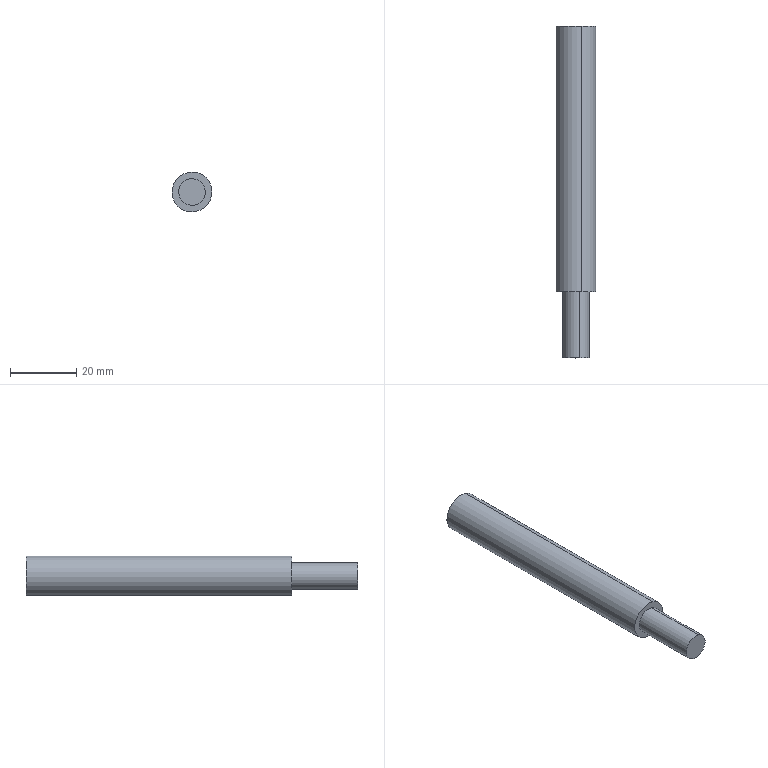Component | SolidWorks | WristClampingPistonRod-2 | 1 solid | 7 faces | box 12 x 100 x 12 mm | volume 10053 mm3 | cylinder 4 | plane 3 | commonest cylinder face diameters 8 x2 12 x2
build123d program:
from build123d import *

# Parameters (mm, degrees)
SKETCH1_R           = 6
BOSS_EXTRUDE1_DEPTH = 80
SKETCH2_R           = 4
BOSS_EXTRUDE2_DEPTH = 20


with BuildPart() as part:
    # Sketch1 → Boss-Extrude1 (new body)
    with BuildSketch(Plane(origin=(0, 0, 0), x_dir=(1, 0, 0), z_dir=(0, 1, 0))):
        with Locations(Location((0, 0, 0), (0, 0, 270))):
            Circle(SKETCH1_R)
    extrude(amount=BOSS_EXTRUDE1_DEPTH)

    # Sketch2 → Boss-Extrude2 (add)
    with BuildSketch(Plane(origin=(0, 80, 0), x_dir=(1, 0, 0), z_dir=(0, 1, 0))):
        with Locations(Location((0, 0, 0), (0, 0, 270))):
            Circle(SKETCH2_R)
    extrude(amount=BOSS_EXTRUDE2_DEPTH)


solid = part.part

# Placed as in the assembly
solid = solid.moved(Location((-125.042, 856.966, 1109.753), (180, 0, 0)))
STEP:
#1=COLOUR_RGB('',0.7922,0.8196,0.9333);
#2=FILL_AREA_STYLE_COLOUR('',#1);
#3=FILL_AREA_STYLE('',(#2));
#4=SURFACE_STYLE_FILL_AREA(#3);
#5=SURFACE_SIDE_STYLE('',(#4));
#6=SURFACE_STYLE_USAGE(.BOTH.,#5);
#7=PRESENTATION_STYLE_ASSIGNMENT((#6));
#8=CARTESIAN_POINT('',(-4.876,29.802,43.841));
#9=VERTEX_POINT('',#8);
#10=CARTESIAN_POINT('',(-4.97,29.802,43.541));
#11=VERTEX_POINT('',#10);
#12=CARTESIAN_POINT('',(-4.923,29.802,43.691));
#13=DIRECTION('',(0.,-1.,0.));
#14=DIRECTION('',(0.2992,0.,0.9542));
#15=AXIS2_PLACEMENT_3D('',#12,#13,#14);
#16=CIRCLE('',#15,0.1575);
#17=EDGE_CURVE('',#9,#11,#16,.T.);
#18=ORIENTED_EDGE('',*,*,#17,.F.);
#19=CARTESIAN_POINT('',(-4.876,30.589,43.841));
#20=VERTEX_POINT('',#19);
#21=CARTESIAN_POINT('',(-4.876,29.802,43.841));
#22=DIRECTION('',(0.,1.,0.));
#23=VECTOR('',#22,39.37);
#24=LINE('',#21,#23);
#25=EDGE_CURVE('',#9,#20,#24,.T.);
#26=ORIENTED_EDGE('',*,*,#25,.T.);
#27=CARTESIAN_POINT('',(-4.97,30.589,43.541));
#28=VERTEX_POINT('',#27);
#29=CARTESIAN_POINT('',(-4.923,30.589,43.691));
#30=DIRECTION('',(0.,-1.,0.));
#31=DIRECTION('',(0.2992,0.,0.9542));
#32=AXIS2_PLACEMENT_3D('',#29,#30,#31);
#33=CIRCLE('',#32,0.1575);
#34=EDGE_CURVE('',#20,#28,#33,.T.);
#35=ORIENTED_EDGE('',*,*,#34,.T.);
#36=CARTESIAN_POINT('',(-4.97,29.802,43.541));
#37=DIRECTION('',(0.,1.,0.));
#38=VECTOR('',#37,39.37);
#39=LINE('',#36,#38);
#40=EDGE_CURVE('',#11,#28,#39,.T.);
#41=ORIENTED_EDGE('',*,*,#40,.F.);
#42=EDGE_LOOP('',(#18,#26,#35,#41));
#43=FACE_OUTER_BOUND('',#42,.T.);
#44=CARTESIAN_POINT('',(-4.923,29.802,43.691));
#45=DIRECTION('',(0.,1.,0.));
#46=DIRECTION('',(-0.2992,0.,-0.9542));
#47=AXIS2_PLACEMENT_3D('',#44,#45,#46);
#48=CYLINDRICAL_SURFACE('',#47,0.1575);
#49=ADVANCED_FACE('',(#43),#48,.T.);
#50=CARTESIAN_POINT('',(-4.852,30.589,43.916));
#51=VERTEX_POINT('',#50);
#52=CARTESIAN_POINT('',(-4.994,30.589,43.466));
#53=VERTEX_POINT('',#52);
#54=CARTESIAN_POINT('',(-4.923,30.589,43.691));
#55=DIRECTION('',(0.,-1.,0.));
#56=DIRECTION('',(0.2992,0.,0.9542));
#57=AXIS2_PLACEMENT_3D('',#54,#55,#56);
#58=CIRCLE('',#57,0.2362);
#59=EDGE_CURVE('',#51,#53,#58,.T.);
#60=ORIENTED_EDGE('',*,*,#59,.F.);
#61=CARTESIAN_POINT('',(-4.852,33.739,43.916));
#62=VERTEX_POINT('',#61);
#63=CARTESIAN_POINT('',(-4.852,30.589,43.916));
#64=DIRECTION('',(0.,1.,0.));
#65=VECTOR('',#64,39.37);
#66=LINE('',#63,#65);
#67=EDGE_CURVE('',#51,#62,#66,.T.);
#68=ORIENTED_EDGE('',*,*,#67,.T.);
#69=CARTESIAN_POINT('',(-4.994,33.739,43.466));
#70=VERTEX_POINT('',#69);
#71=CARTESIAN_POINT('',(-4.923,33.739,43.691));
#72=DIRECTION('',(0.,-1.,0.));
#73=DIRECTION('',(0.2992,0.,0.9542));
#74=AXIS2_PLACEMENT_3D('',#71,#72,#73);
#75=CIRCLE('',#74,0.2362);
#76=EDGE_CURVE('',#62,#70,#75,.T.);
#77=ORIENTED_EDGE('',*,*,#76,.T.);
#78=CARTESIAN_POINT('',(-4.994,30.589,43.466));
#79=DIRECTION('',(0.,1.,0.));
#80=VECTOR('',#79,39.37);
#81=LINE('',#78,#80);
#82=EDGE_CURVE('',#53,#70,#81,.T.);
#83=ORIENTED_EDGE('',*,*,#82,.F.);
#84=EDGE_LOOP('',(#60,#68,#77,#83));
#85=FACE_OUTER_BOUND('',#84,.T.);
#86=CARTESIAN_POINT('',(-4.923,30.589,43.691));
#87=DIRECTION('',(0.,1.,0.));
#88=DIRECTION('',(-0.2992,0.,-0.9542));
#89=AXIS2_PLACEMENT_3D('',#86,#87,#88);
#90=CYLINDRICAL_SURFACE('',#89,0.2362);
#91=ADVANCED_FACE('',(#85),#90,.T.);
#92=ORIENTED_EDGE('',*,*,#67,.F.);
#93=CARTESIAN_POINT('',(-4.923,30.589,43.691));
#94=DIRECTION('',(0.,-1.,0.));
#95=DIRECTION('',(0.2992,0.,0.9542));
#96=AXIS2_PLACEMENT_3D('',#93,#94,#95);
#97=CIRCLE('',#96,0.2362);
#98=EDGE_CURVE('',#53,#51,#97,.T.);
#99=ORIENTED_EDGE('',*,*,#98,.F.);
#100=ORIENTED_EDGE('',*,*,#82,.T.);
#101=CARTESIAN_POINT('',(-4.923,33.739,43.691));
#102=DIRECTION('',(0.,-1.,0.));
#103=DIRECTION('',(0.2992,0.,0.9542));
#104=AXIS2_PLACEMENT_3D('',#101,#102,#103);
#105=CIRCLE('',#104,0.2362);
#106=EDGE_CURVE('',#70,#62,#105,.T.);
#107=ORIENTED_EDGE('',*,*,#106,.T.);
#108=EDGE_LOOP('',(#92,#99,#100,#107));
#109=FACE_OUTER_BOUND('',#108,.T.);
#110=CARTESIAN_POINT('',(-4.923,30.589,43.691));
#111=DIRECTION('',(0.,1.,0.));
#112=DIRECTION('',(-0.2992,0.,-0.9542));
#113=AXIS2_PLACEMENT_3D('',#110,#111,#112);
#114=CYLINDRICAL_SURFACE('',#113,0.2362);
#115=ADVANCED_FACE('',(#109),#114,.T.);
#116=CARTESIAN_POINT('',(-4.923,30.589,43.691));
#117=DIRECTION('',(0.,-1.,0.));
#118=DIRECTION('',(0.2992,0.,0.9542));
#119=AXIS2_PLACEMENT_3D('',#116,#117,#118);
#120=CIRCLE('',#119,0.1575);
#121=EDGE_CURVE('',#28,#20,#120,.T.);
#122=ORIENTED_EDGE('',*,*,#121,.F.);
#123=ORIENTED_EDGE('',*,*,#34,.F.);
#124=EDGE_LOOP('',(#122,#123));
#125=FACE_BOUND('',#124,.T.);
#126=ORIENTED_EDGE('',*,*,#98,.T.);
#127=ORIENTED_EDGE('',*,*,#59,.T.);
#128=EDGE_LOOP('',(#126,#127));
#129=FACE_OUTER_BOUND('',#128,.T.);
#130=CARTESIAN_POINT('',(-4.923,30.589,43.691));
#131=DIRECTION('',(0.,-1.,0.));
#132=DIRECTION('',(0.2992,0.,0.9542));
#133=AXIS2_PLACEMENT_3D('',#130,#131,#132);
#134=PLANE('',#133);
#135=ADVANCED_FACE('',(#125,#129),#134,.T.);
#136=ORIENTED_EDGE('',*,*,#106,.F.);
#137=ORIENTED_EDGE('',*,*,#76,.F.);
#138=EDGE_LOOP('',(#136,#137));
#139=FACE_OUTER_BOUND('',#138,.T.);
#140=CARTESIAN_POINT('',(-4.923,33.739,43.691));
#141=DIRECTION('',(0.,-1.,0.));
#142=DIRECTION('',(0.2992,0.,0.9542));
#143=AXIS2_PLACEMENT_3D('',#140,#141,#142);
#144=PLANE('',#143);
#145=ADVANCED_FACE('',(#139),#144,.F.);
#146=ORIENTED_EDGE('',*,*,#25,.F.);
#147=CARTESIAN_POINT('',(-4.923,29.802,43.691));
#148=DIRECTION('',(0.,-1.,0.));
#149=DIRECTION('',(0.2992,0.,0.9542));
#150=AXIS2_PLACEMENT_3D('',#147,#148,#149);
#151=CIRCLE('',#150,0.1575);
#152=EDGE_CURVE('',#11,#9,#151,.T.);
#153=ORIENTED_EDGE('',*,*,#152,.F.);
#154=ORIENTED_EDGE('',*,*,#40,.T.);
#155=ORIENTED_EDGE('',*,*,#121,.T.);
#156=EDGE_LOOP('',(#146,#153,#154,#155));
#157=FACE_OUTER_BOUND('',#156,.T.);
#158=CARTESIAN_POINT('',(-4.923,29.802,43.691));
#159=DIRECTION('',(0.,1.,0.));
#160=DIRECTION('',(-0.2992,0.,-0.9542));
#161=AXIS2_PLACEMENT_3D('',#158,#159,#160);
#162=CYLINDRICAL_SURFACE('',#161,0.1575);
#163=ADVANCED_FACE('',(#157),#162,.T.);
#164=ORIENTED_EDGE('',*,*,#152,.T.);
#165=ORIENTED_EDGE('',*,*,#17,.T.);
#166=EDGE_LOOP('',(#164,#165));
#167=FACE_OUTER_BOUND('',#166,.T.);
#168=CARTESIAN_POINT('',(-4.923,29.802,43.691));
#169=DIRECTION('',(0.,-1.,0.));
#170=DIRECTION('',(0.2992,0.,0.9542));
#171=AXIS2_PLACEMENT_3D('',#168,#169,#170);
#172=PLANE('',#171);
#173=ADVANCED_FACE('',(#167),#172,.T.);
#174=CLOSED_SHELL('',(#49,#91,#115,#135,#145,#163,#173));
#175=MANIFOLD_SOLID_BREP('',#174);
#176=STYLED_ITEM('',(#7),#175);
#177=PRESENTATION_LAYER_ASSIGNMENT('','',(#176));
#178=(LENGTH_UNIT()NAMED_UNIT(*)SI_UNIT($,.METRE.));
#179=LENGTH_MEASURE_WITH_UNIT(LENGTH_MEASURE(0.0254),#178);
#180=DIMENSIONAL_EXPONENTS(1.,0.,0.,0.,0.,0.,0.);
#181=(CONVERSION_BASED_UNIT('',#179)LENGTH_UNIT()NAMED_UNIT(#180));
#182=UNCERTAINTY_MEASURE_WITH_UNIT(LENGTH_MEASURE(0.00001),#181,'','');
#183=(NAMED_UNIT(*)PLANE_ANGLE_UNIT()SI_UNIT($,.RADIAN.));
#184=(NAMED_UNIT(*)SI_UNIT($,.STERADIAN.)SOLID_ANGLE_UNIT());
#185=(GEOMETRIC_REPRESENTATION_CONTEXT(3)GLOBAL_UNCERTAINTY_ASSIGNED_CONTEXT((#182))GLOBAL_UNIT_ASSIGNED_CONTEXT((#181,#183,#184))REPRESENTATION_CONTEXT('',''));
#186=MECHANICAL_DESIGN_GEOMETRIC_PRESENTATION_REPRESENTATION('',(#176),#185);
#187=CARTESIAN_POINT('',(0.,0.,0.));
#188=DIRECTION('',(0.,0.,1.));
#189=DIRECTION('',(1.,0.,0.));
#190=AXIS2_PLACEMENT_3D('',#187,#188,#189);
#191=(LENGTH_UNIT()NAMED_UNIT(*)SI_UNIT($,.METRE.));
#192=LENGTH_MEASURE_WITH_UNIT(LENGTH_MEASURE(0.0254),#191);
#193=DIMENSIONAL_EXPONENTS(1.,0.,0.,0.,0.,0.,0.);
#194=(CONVERSION_BASED_UNIT('',#192)LENGTH_UNIT()NAMED_UNIT(#193));
#195=UNCERTAINTY_MEASURE_WITH_UNIT(LENGTH_MEASURE(0.00001),#194,'','');
#196=(NAMED_UNIT(*)PLANE_ANGLE_UNIT()SI_UNIT($,.RADIAN.));
#197=(NAMED_UNIT(*)SI_UNIT($,.STERADIAN.)SOLID_ANGLE_UNIT());
#198=(GEOMETRIC_REPRESENTATION_CONTEXT(3)GLOBAL_UNCERTAINTY_ASSIGNED_CONTEXT((#195))GLOBAL_UNIT_ASSIGNED_CONTEXT((#194,#196,#197))REPRESENTATION_CONTEXT('',''));
#199=ADVANCED_BREP_SHAPE_REPRESENTATION('',(#175,#190),#198);